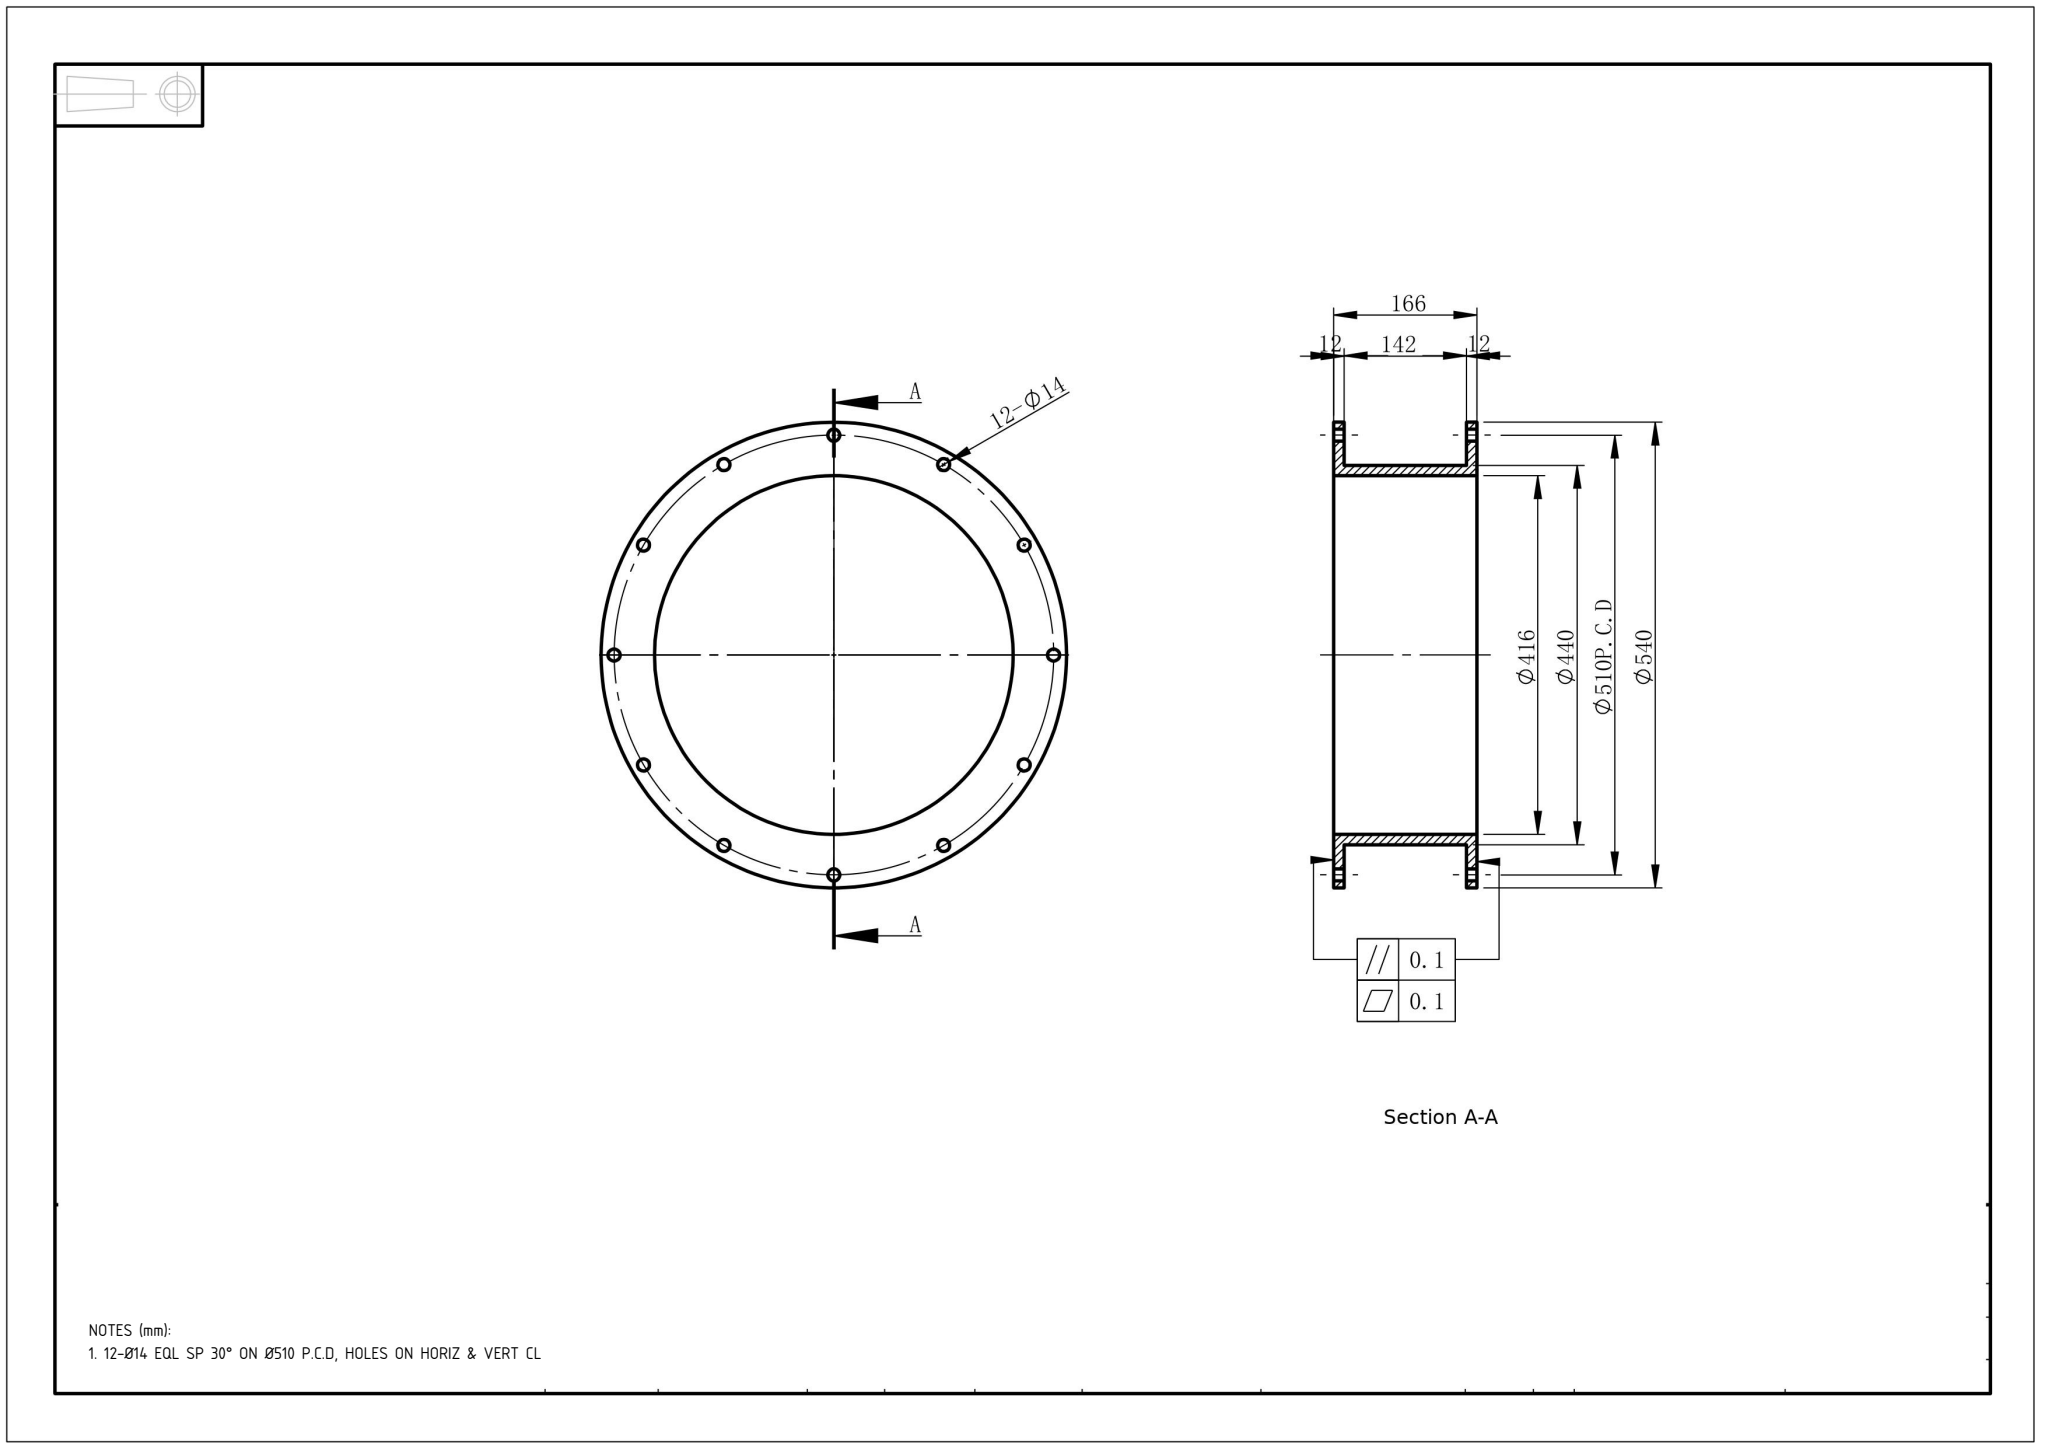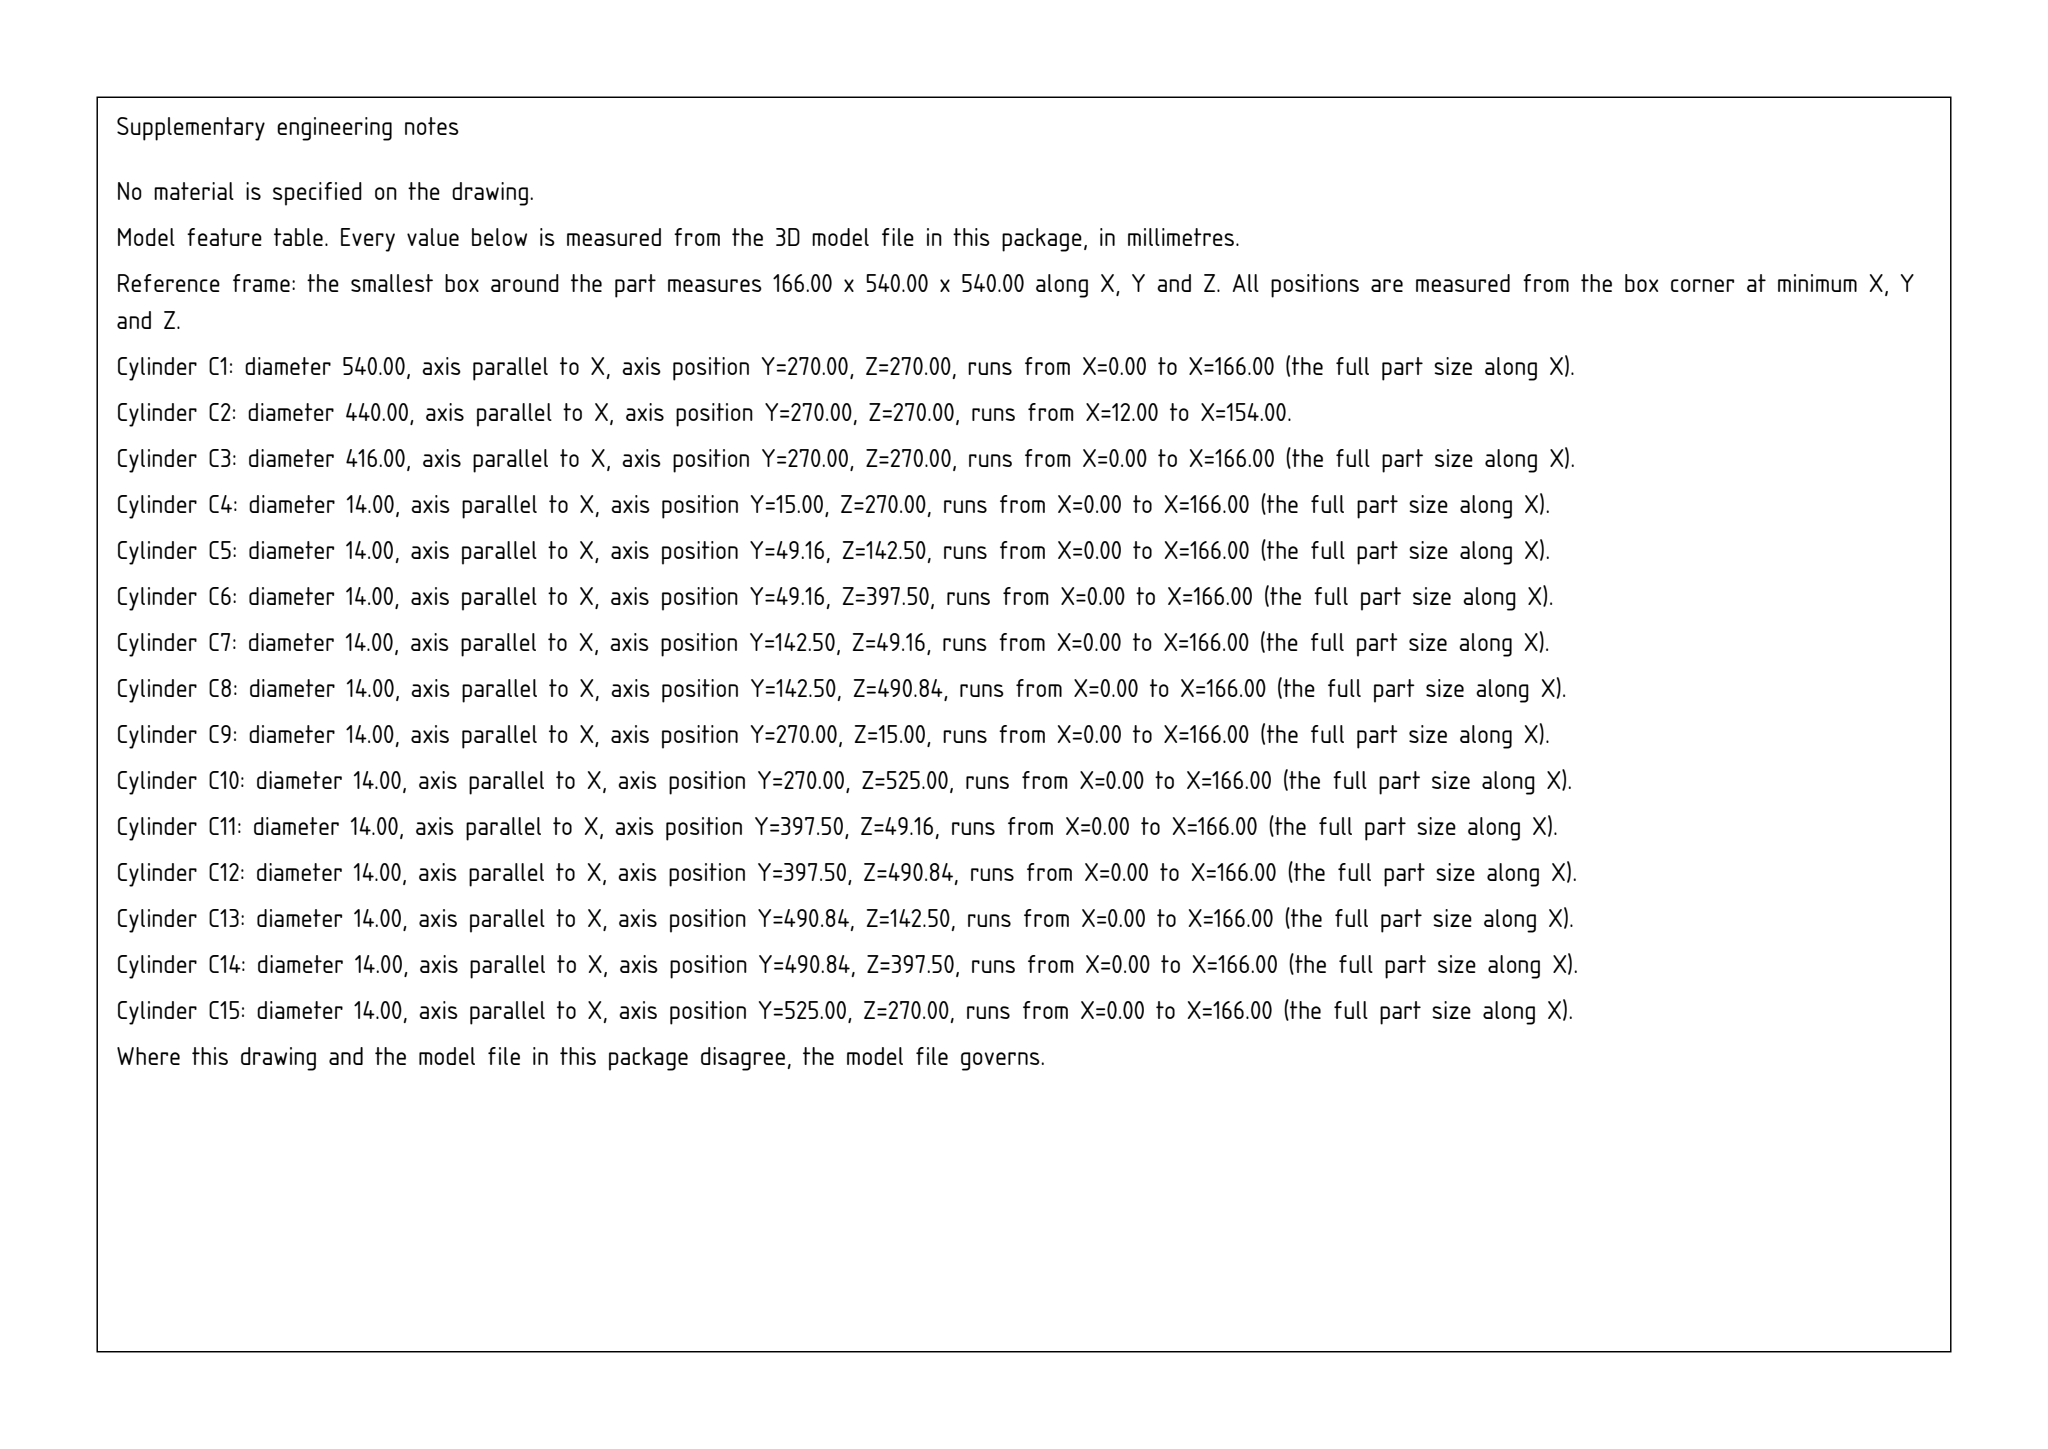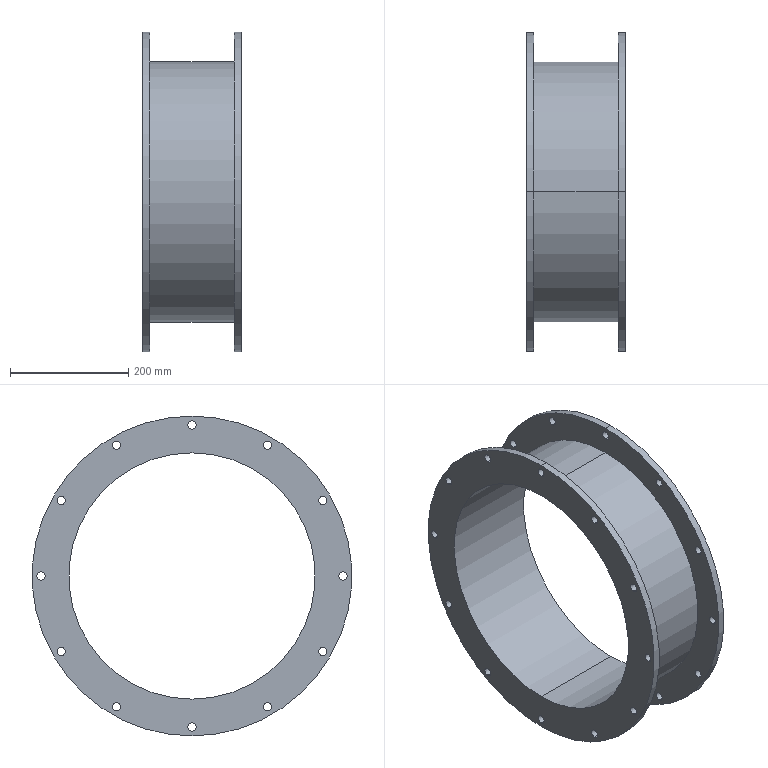Part | SolidWorks | mm | 1 solid | 60 faces | box 166 x 540 x 540 mm | volume 4481369 mm3 | cylinder 56 | plane 4 | commonest cylinder face diameters 14 x48 540 x4 440 x2 416 x2
Drawing notes:
12-Ø14 EQL SP 30° ON Ø510 P.C.D, HOLES ON HORIZ & VERT CL | from the solid: 12 Ø14 holes at R255 from axis (270,270); positions (15,270),(49.16,142.5),(142.5,49.16),(270,15),(397.5,49.16),(490.84,142.5),(525,270),(490.84,397.5),(397.5,490.84),(270,525),(142.5,490.84),(49.16,397.5) = 30° increments starting on centerlines
build123d program:
from build123d import *

# Parameters (mm, degrees)
SKETCH3_R          = 7
CUT_EXTRUDE1_DEPTH = 417.36
CIRPATTERN1_COUNT  = 12


with BuildPart() as part:
    # Sketch1 → Revolve1 (revolve)
    with BuildSketch(Plane.XY, mode=Mode.PRIVATE) as revolve1_sk:
        Polygon((-83, 208), (-83, 270), (-71, 270), (-71, 220), (71, 220), (71, 270), (83, 270), (83, 208), align=None)
    revolve(revolve1_sk.sketch.rotate(Axis((-1000, 0, 0), (1, 0, 0)), 90), axis=Axis((-1000, 0, 0), (1, 0, 0)))

    # Sketch3 → Cut-Extrude1 (cut, through all)
    with BuildSketch(Plane.ZY.offset(83)):
        with Locations((0, 255)):
            Circle(SKETCH3_R)
    cut_extrude1 = extrude(amount=-CUT_EXTRUDE1_DEPTH, mode=Mode.SUBTRACT)

    # CirPattern1: Cut-Extrude1 ×12 about axis
    cirpattern1_axis = Axis((0, 0, 0), (1, 0, 0))
    for i in range(1, CIRPATTERN1_COUNT):
        add(cut_extrude1.rotate(cirpattern1_axis, i * 360 / CIRPATTERN1_COUNT), mode=Mode.SUBTRACT)


solid = part.part